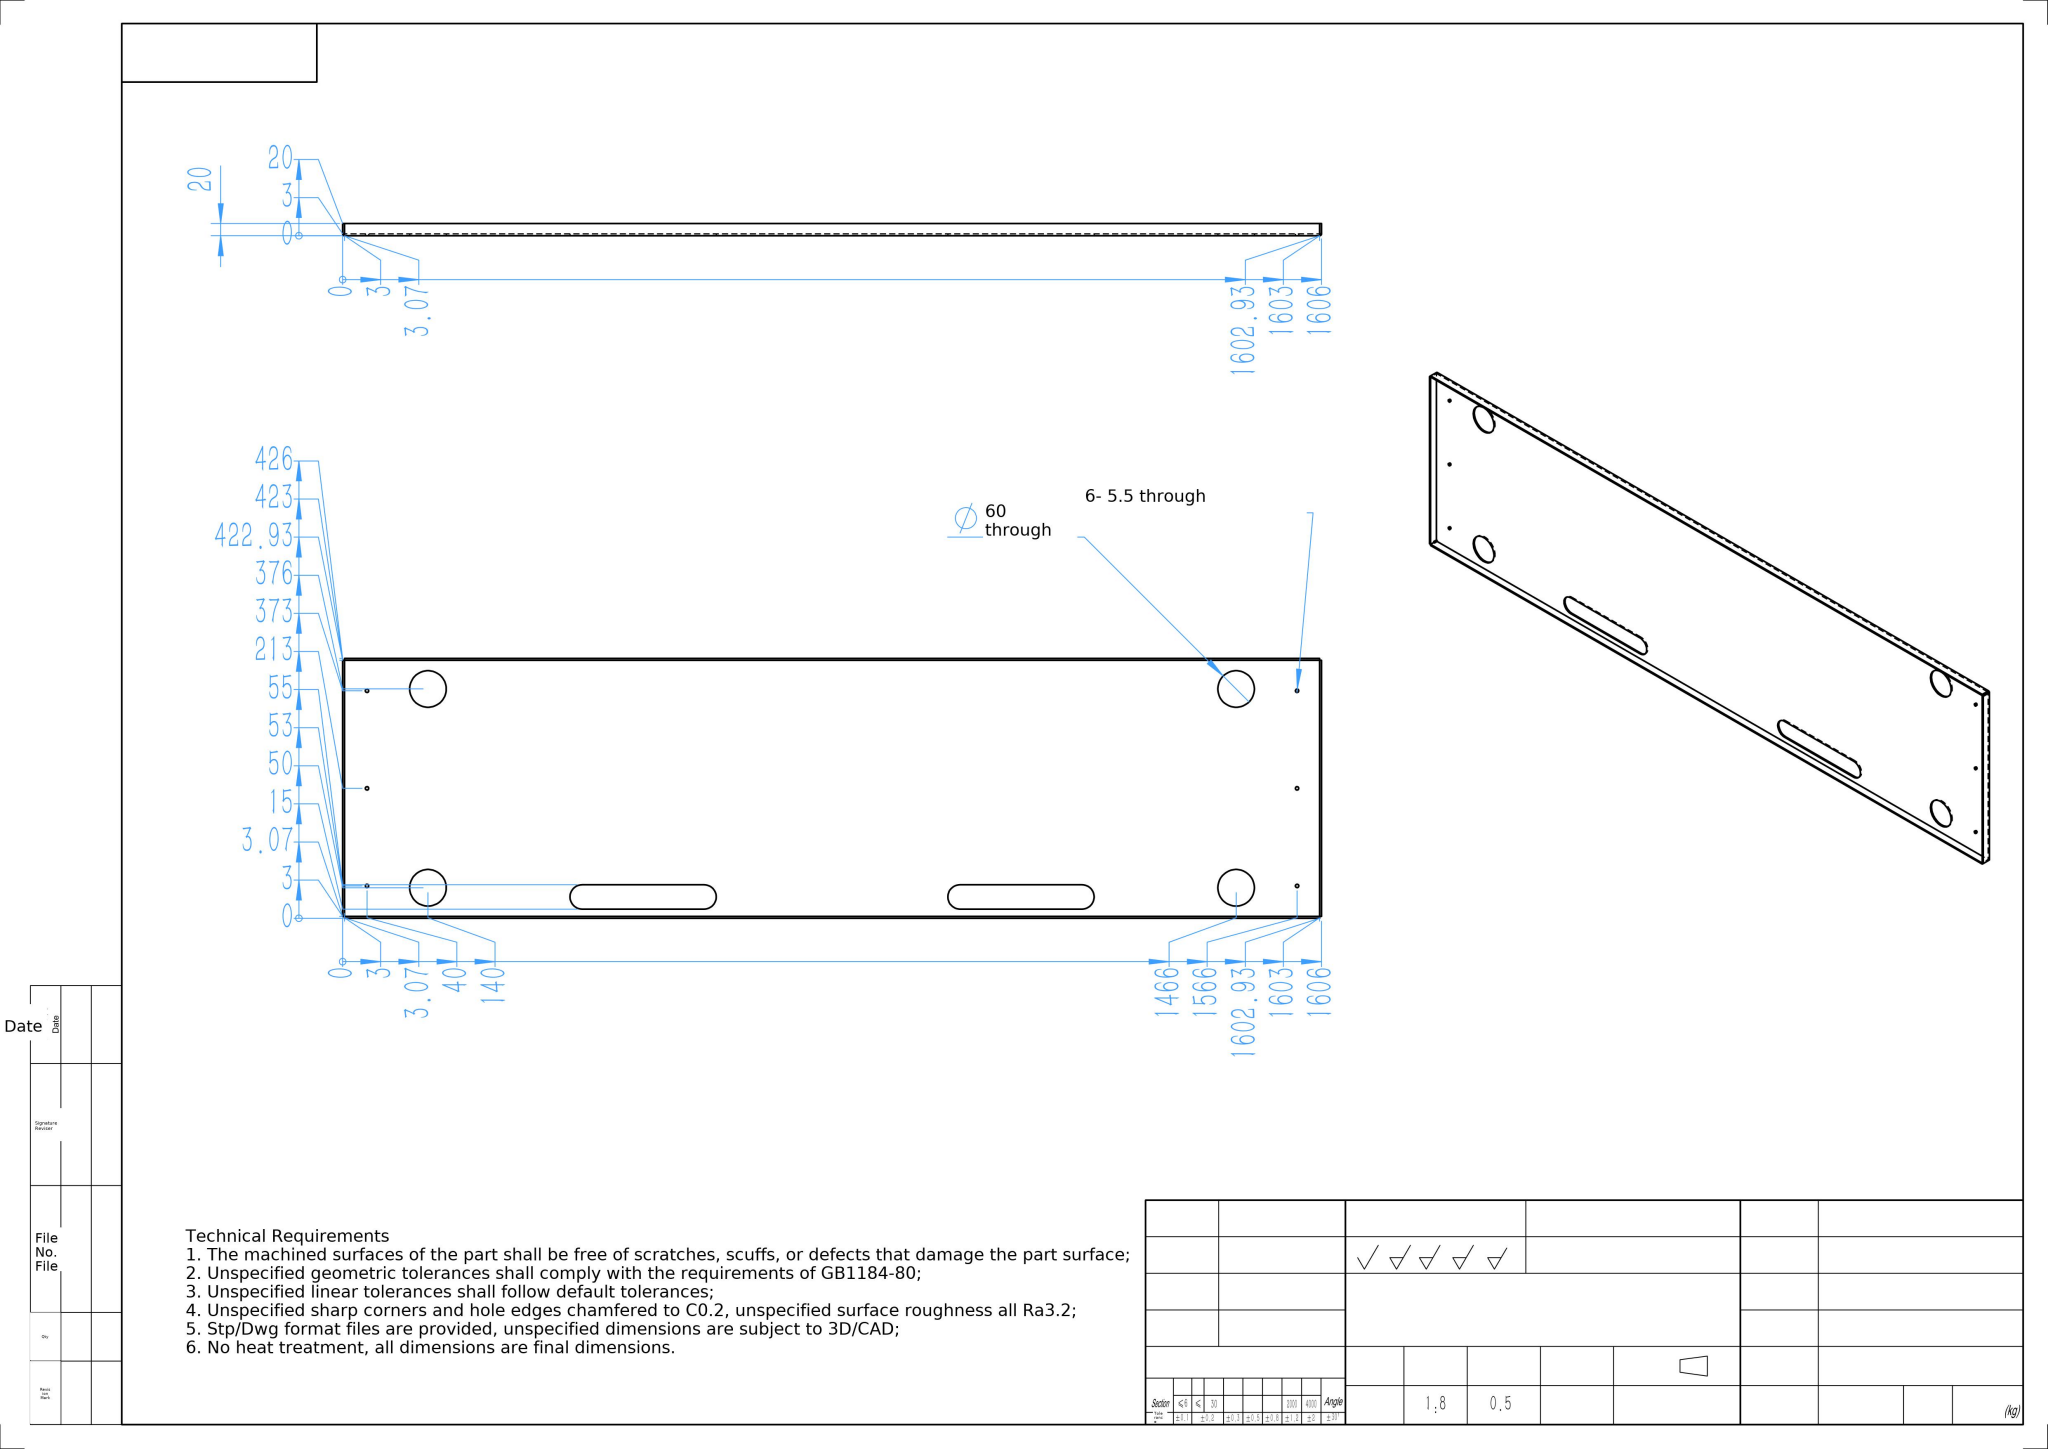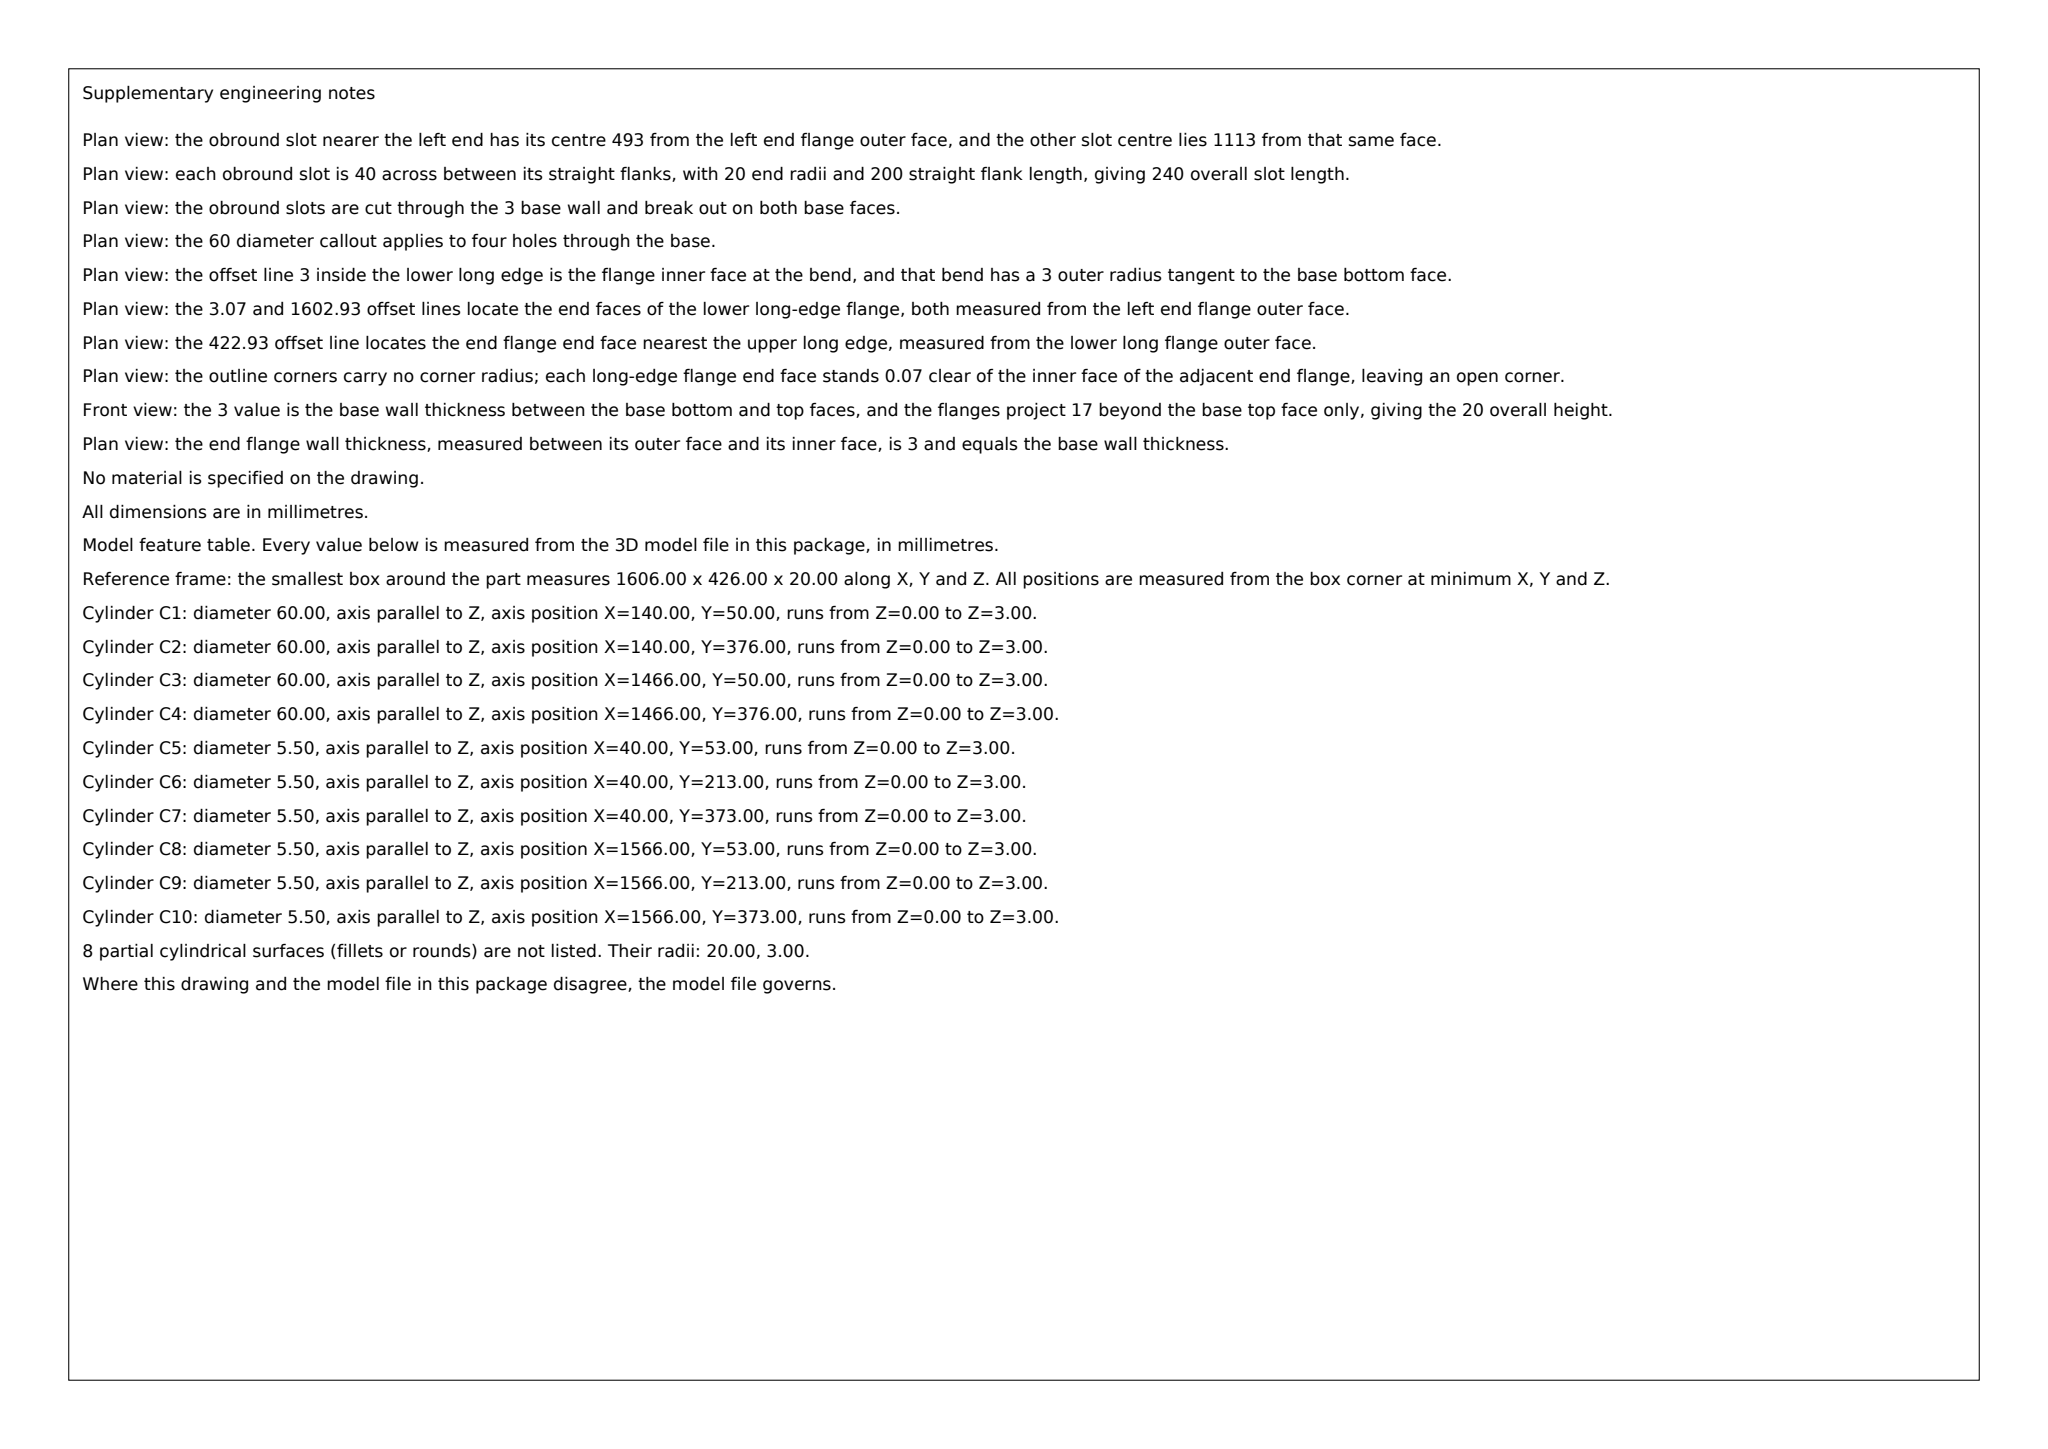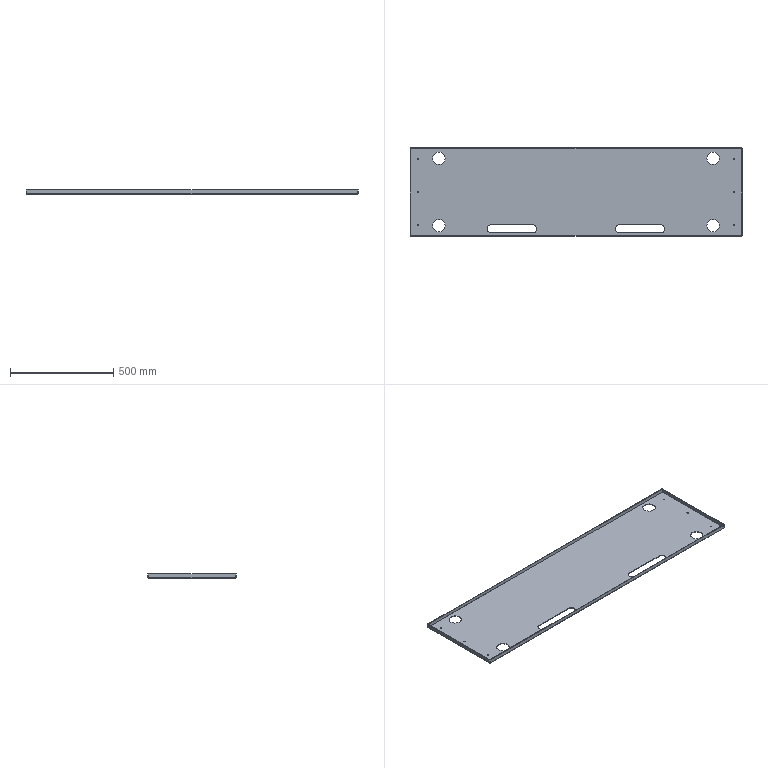Part | SolidWorks | mm | 1 solid | 64 faces | box 1606 x 426 x 20 mm | volume 2160659 mm3 | cylinder 30 | plane 26 | spline 8 | commonest cylinder face diameters 5.5 x12 60 x8 40 x6 6 x4